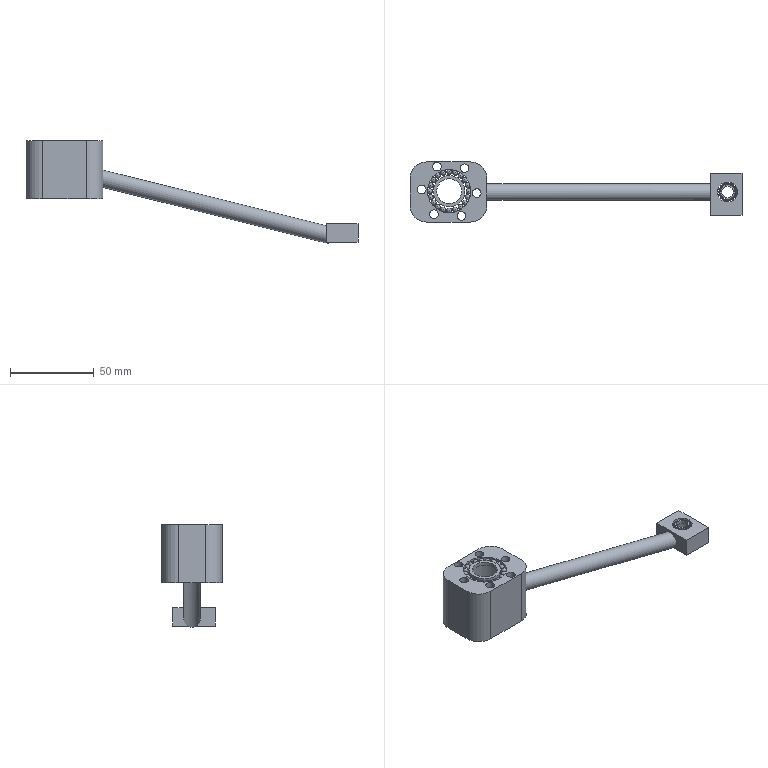Component | NX | RED | 23 solids | 74 faces | volume 47061 mm3 | sphere 40 | cylinder 17 | plane 17 | commonest cylinder face diameters 5.213 x6 20 x4 8.686 x1 7.019 x1 10 x1 26 x1 11.939 x1 18.889 x1